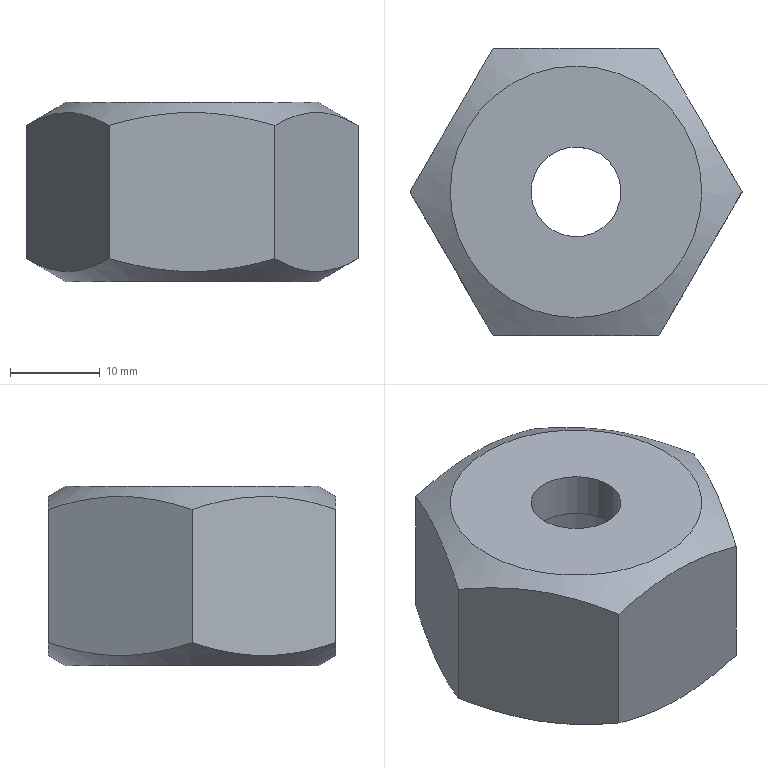Component | NX | GLAND_NUT | 1 solid | 15 faces | volume 9419 mm3 | plane 10 | cylinder 3 | cone 2 | commonest cylinder face diameters 24 x1 28 x1 10 x1